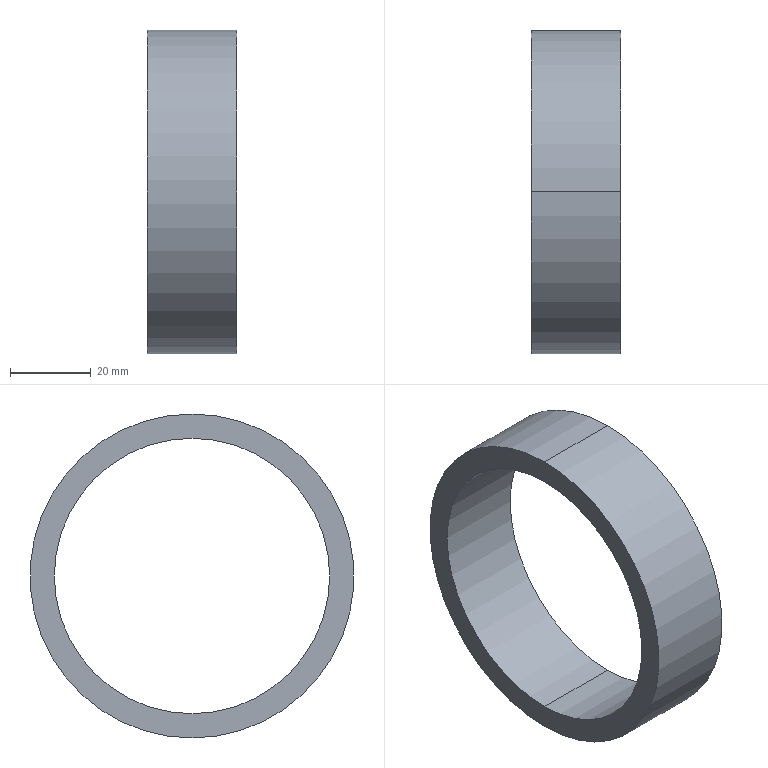Component | SolidWorks | 3CopperRing-1 | 1 solid | 6 faces | box 22 x 80 x 80 mm | volume 30687 mm3 | cylinder 4 | plane 2 | commonest cylinder face diameters 68 x2 80 x2
build123d program:
from build123d import *

# Parameters (mm, degrees)
SKETCH19_R          = 40
SKETCH19_R_2        = 34
BOSS_EXTRUDE6_DEPTH = 22


with BuildPart() as part:
    # Sketch19 → Boss-Extrude6 (new body)
    with BuildSketch(Plane(origin=(0, 0, 0), x_dir=(1, 0, 0), z_dir=(0, 1, 0))):
        with Locations(Location((0, 0, 0), (0, 0, 270))):
            Circle(SKETCH19_R)
        with Locations(Location((0, 0, 0), (0, 0, 270))):
            Circle(SKETCH19_R_2, mode=Mode.SUBTRACT)
    extrude(amount=BOSS_EXTRUDE6_DEPTH)


solid = part.part

# Placed as in the assembly
solid = solid.moved(Location((70.957, 1.776, 250), (0, 0, 90)))
STEP:
#1=COLOUR_RGB('',0.7922,0.8196,0.9333);
#2=FILL_AREA_STYLE_COLOUR('',#1);
#3=FILL_AREA_STYLE('',(#2));
#4=SURFACE_STYLE_FILL_AREA(#3);
#5=SURFACE_SIDE_STYLE('',(#4));
#6=SURFACE_STYLE_USAGE(.BOTH.,#5);
#7=PRESENTATION_STYLE_ASSIGNMENT((#6));
#8=CARTESIAN_POINT('',(1.927,0.06992,8.504));
#9=VERTEX_POINT('',#8);
#10=CARTESIAN_POINT('',(1.927,0.06992,11.181));
#11=VERTEX_POINT('',#10);
#12=CARTESIAN_POINT('',(1.927,0.06992,9.843));
#13=DIRECTION('',(-1.,-0.,-0.));
#14=DIRECTION('',(0.,-0.,1.));
#15=AXIS2_PLACEMENT_3D('',#12,#13,#14);
#16=CIRCLE('',#15,1.339);
#17=EDGE_CURVE('',#9,#11,#16,.T.);
#18=ORIENTED_EDGE('',*,*,#17,.T.);
#19=CARTESIAN_POINT('',(2.794,0.06992,11.181));
#20=VERTEX_POINT('',#19);
#21=CARTESIAN_POINT('',(1.927,0.06992,11.181));
#22=DIRECTION('',(1.,0.,0.));
#23=VECTOR('',#22,39.37);
#24=LINE('',#21,#23);
#25=EDGE_CURVE('',#11,#20,#24,.T.);
#26=ORIENTED_EDGE('',*,*,#25,.T.);
#27=CARTESIAN_POINT('',(2.794,0.06992,8.504));
#28=VERTEX_POINT('',#27);
#29=CARTESIAN_POINT('',(2.794,0.06992,9.843));
#30=DIRECTION('',(-1.,-0.,-0.));
#31=DIRECTION('',(0.,-0.,1.));
#32=AXIS2_PLACEMENT_3D('',#29,#30,#31);
#33=CIRCLE('',#32,1.339);
#34=EDGE_CURVE('',#28,#20,#33,.T.);
#35=ORIENTED_EDGE('',*,*,#34,.F.);
#36=CARTESIAN_POINT('',(1.927,0.06992,8.504));
#37=DIRECTION('',(1.,0.,0.));
#38=VECTOR('',#37,39.37);
#39=LINE('',#36,#38);
#40=EDGE_CURVE('',#9,#28,#39,.T.);
#41=ORIENTED_EDGE('',*,*,#40,.F.);
#42=EDGE_LOOP('',(#18,#26,#35,#41));
#43=FACE_OUTER_BOUND('',#42,.T.);
#44=CARTESIAN_POINT('',(1.927,0.06992,9.843));
#45=DIRECTION('',(1.,0.,0.));
#46=DIRECTION('',(0.,0.,-1.));
#47=AXIS2_PLACEMENT_3D('',#44,#45,#46);
#48=CYLINDRICAL_SURFACE('',#47,1.339);
#49=ADVANCED_FACE('',(#43),#48,.F.);
#50=CARTESIAN_POINT('',(1.927,0.06992,11.417));
#51=VERTEX_POINT('',#50);
#52=CARTESIAN_POINT('',(1.927,0.06992,8.268));
#53=VERTEX_POINT('',#52);
#54=CARTESIAN_POINT('',(1.927,0.06992,9.843));
#55=DIRECTION('',(-1.,-0.,-0.));
#56=DIRECTION('',(0.,-0.,1.));
#57=AXIS2_PLACEMENT_3D('',#54,#55,#56);
#58=CIRCLE('',#57,1.575);
#59=EDGE_CURVE('',#51,#53,#58,.T.);
#60=ORIENTED_EDGE('',*,*,#59,.F.);
#61=CARTESIAN_POINT('',(2.794,0.06992,11.417));
#62=VERTEX_POINT('',#61);
#63=CARTESIAN_POINT('',(1.927,0.06992,11.417));
#64=DIRECTION('',(1.,0.,0.));
#65=VECTOR('',#64,39.37);
#66=LINE('',#63,#65);
#67=EDGE_CURVE('',#51,#62,#66,.T.);
#68=ORIENTED_EDGE('',*,*,#67,.T.);
#69=CARTESIAN_POINT('',(2.794,0.06992,8.268));
#70=VERTEX_POINT('',#69);
#71=CARTESIAN_POINT('',(2.794,0.06992,9.843));
#72=DIRECTION('',(-1.,-0.,-0.));
#73=DIRECTION('',(0.,-0.,1.));
#74=AXIS2_PLACEMENT_3D('',#71,#72,#73);
#75=CIRCLE('',#74,1.575);
#76=EDGE_CURVE('',#62,#70,#75,.T.);
#77=ORIENTED_EDGE('',*,*,#76,.T.);
#78=CARTESIAN_POINT('',(1.927,0.06992,8.268));
#79=DIRECTION('',(1.,0.,0.));
#80=VECTOR('',#79,39.37);
#81=LINE('',#78,#80);
#82=EDGE_CURVE('',#53,#70,#81,.T.);
#83=ORIENTED_EDGE('',*,*,#82,.F.);
#84=EDGE_LOOP('',(#60,#68,#77,#83));
#85=FACE_OUTER_BOUND('',#84,.T.);
#86=CARTESIAN_POINT('',(1.927,0.06992,9.843));
#87=DIRECTION('',(1.,0.,0.));
#88=DIRECTION('',(0.,0.,-1.));
#89=AXIS2_PLACEMENT_3D('',#86,#87,#88);
#90=CYLINDRICAL_SURFACE('',#89,1.575);
#91=ADVANCED_FACE('',(#85),#90,.T.);
#92=CARTESIAN_POINT('',(1.927,0.06992,9.843));
#93=DIRECTION('',(-1.,-0.,-0.));
#94=DIRECTION('',(0.,-0.,1.));
#95=AXIS2_PLACEMENT_3D('',#92,#93,#94);
#96=CIRCLE('',#95,1.575);
#97=EDGE_CURVE('',#53,#51,#96,.T.);
#98=ORIENTED_EDGE('',*,*,#97,.T.);
#99=ORIENTED_EDGE('',*,*,#59,.T.);
#100=EDGE_LOOP('',(#98,#99));
#101=FACE_OUTER_BOUND('',#100,.T.);
#102=ORIENTED_EDGE('',*,*,#17,.F.);
#103=CARTESIAN_POINT('',(1.927,0.06992,9.843));
#104=DIRECTION('',(-1.,-0.,-0.));
#105=DIRECTION('',(0.,-0.,1.));
#106=AXIS2_PLACEMENT_3D('',#103,#104,#105);
#107=CIRCLE('',#106,1.339);
#108=EDGE_CURVE('',#11,#9,#107,.T.);
#109=ORIENTED_EDGE('',*,*,#108,.F.);
#110=EDGE_LOOP('',(#102,#109));
#111=FACE_BOUND('',#110,.T.);
#112=CARTESIAN_POINT('',(1.927,0.06992,9.843));
#113=DIRECTION('',(-1.,-0.,-0.));
#114=DIRECTION('',(-0.,-0.,1.));
#115=AXIS2_PLACEMENT_3D('',#112,#113,#114);
#116=PLANE('',#115);
#117=ADVANCED_FACE('',(#101,#111),#116,.T.);
#118=CARTESIAN_POINT('',(2.794,0.06992,9.843));
#119=DIRECTION('',(-1.,-0.,-0.));
#120=DIRECTION('',(0.,-0.,1.));
#121=AXIS2_PLACEMENT_3D('',#118,#119,#120);
#122=CIRCLE('',#121,1.575);
#123=EDGE_CURVE('',#70,#62,#122,.T.);
#124=ORIENTED_EDGE('',*,*,#123,.F.);
#125=ORIENTED_EDGE('',*,*,#76,.F.);
#126=EDGE_LOOP('',(#124,#125));
#127=FACE_OUTER_BOUND('',#126,.T.);
#128=ORIENTED_EDGE('',*,*,#34,.T.);
#129=CARTESIAN_POINT('',(2.794,0.06992,9.843));
#130=DIRECTION('',(-1.,-0.,-0.));
#131=DIRECTION('',(0.,-0.,1.));
#132=AXIS2_PLACEMENT_3D('',#129,#130,#131);
#133=CIRCLE('',#132,1.339);
#134=EDGE_CURVE('',#20,#28,#133,.T.);
#135=ORIENTED_EDGE('',*,*,#134,.T.);
#136=EDGE_LOOP('',(#128,#135));
#137=FACE_BOUND('',#136,.T.);
#138=CARTESIAN_POINT('',(2.794,0.06992,9.843));
#139=DIRECTION('',(-1.,-0.,-0.));
#140=DIRECTION('',(-0.,-0.,1.));
#141=AXIS2_PLACEMENT_3D('',#138,#139,#140);
#142=PLANE('',#141);
#143=ADVANCED_FACE('',(#127,#137),#142,.F.);
#144=ORIENTED_EDGE('',*,*,#67,.F.);
#145=ORIENTED_EDGE('',*,*,#97,.F.);
#146=ORIENTED_EDGE('',*,*,#82,.T.);
#147=ORIENTED_EDGE('',*,*,#123,.T.);
#148=EDGE_LOOP('',(#144,#145,#146,#147));
#149=FACE_OUTER_BOUND('',#148,.T.);
#150=CARTESIAN_POINT('',(1.927,0.06992,9.843));
#151=DIRECTION('',(1.,0.,0.));
#152=DIRECTION('',(0.,0.,-1.));
#153=AXIS2_PLACEMENT_3D('',#150,#151,#152);
#154=CYLINDRICAL_SURFACE('',#153,1.575);
#155=ADVANCED_FACE('',(#149),#154,.T.);
#156=ORIENTED_EDGE('',*,*,#25,.F.);
#157=ORIENTED_EDGE('',*,*,#108,.T.);
#158=ORIENTED_EDGE('',*,*,#40,.T.);
#159=ORIENTED_EDGE('',*,*,#134,.F.);
#160=EDGE_LOOP('',(#156,#157,#158,#159));
#161=FACE_OUTER_BOUND('',#160,.T.);
#162=CARTESIAN_POINT('',(1.927,0.06992,9.843));
#163=DIRECTION('',(1.,0.,0.));
#164=DIRECTION('',(0.,0.,-1.));
#165=AXIS2_PLACEMENT_3D('',#162,#163,#164);
#166=CYLINDRICAL_SURFACE('',#165,1.339);
#167=ADVANCED_FACE('',(#161),#166,.F.);
#168=CLOSED_SHELL('',(#49,#91,#117,#143,#155,#167));
#169=MANIFOLD_SOLID_BREP('',#168);
#170=STYLED_ITEM('',(#7),#169);
#171=PRESENTATION_LAYER_ASSIGNMENT('','',(#170));
#172=CARTESIAN_POINT('',(0.,0.,0.));
#173=DIRECTION('',(0.,0.,1.));
#174=DIRECTION('',(1.,0.,0.));
#175=AXIS2_PLACEMENT_3D('',#172,#173,#174);
#176=(LENGTH_UNIT()NAMED_UNIT(*)SI_UNIT($,.METRE.));
#177=LENGTH_MEASURE_WITH_UNIT(LENGTH_MEASURE(0.0254),#176);
#178=DIMENSIONAL_EXPONENTS(1.,0.,0.,0.,0.,0.,0.);
#179=(CONVERSION_BASED_UNIT('',#177)LENGTH_UNIT()NAMED_UNIT(#178));
#180=UNCERTAINTY_MEASURE_WITH_UNIT(LENGTH_MEASURE(0.00001),#179,'','');
#181=(NAMED_UNIT(*)PLANE_ANGLE_UNIT()SI_UNIT($,.RADIAN.));
#182=(NAMED_UNIT(*)SI_UNIT($,.STERADIAN.)SOLID_ANGLE_UNIT());
#183=(GEOMETRIC_REPRESENTATION_CONTEXT(3)GLOBAL_UNCERTAINTY_ASSIGNED_CONTEXT((#180))GLOBAL_UNIT_ASSIGNED_CONTEXT((#179,#181,#182))REPRESENTATION_CONTEXT('',''));
#184=ADVANCED_BREP_SHAPE_REPRESENTATION('',(#169,#175),#183);
#185=(LENGTH_UNIT()NAMED_UNIT(*)SI_UNIT($,.METRE.));
#186=LENGTH_MEASURE_WITH_UNIT(LENGTH_MEASURE(0.0254),#185);
#187=DIMENSIONAL_EXPONENTS(1.,0.,0.,0.,0.,0.,0.);
#188=(CONVERSION_BASED_UNIT('',#186)LENGTH_UNIT()NAMED_UNIT(#187));
#189=UNCERTAINTY_MEASURE_WITH_UNIT(LENGTH_MEASURE(0.00001),#188,'','');
#190=(NAMED_UNIT(*)PLANE_ANGLE_UNIT()SI_UNIT($,.RADIAN.));
#191=(NAMED_UNIT(*)SI_UNIT($,.STERADIAN.)SOLID_ANGLE_UNIT());
#192=(GEOMETRIC_REPRESENTATION_CONTEXT(3)GLOBAL_UNCERTAINTY_ASSIGNED_CONTEXT((#189))GLOBAL_UNIT_ASSIGNED_CONTEXT((#188,#190,#191))REPRESENTATION_CONTEXT('',''));
#193=MECHANICAL_DESIGN_GEOMETRIC_PRESENTATION_REPRESENTATION('',(#170),#192);